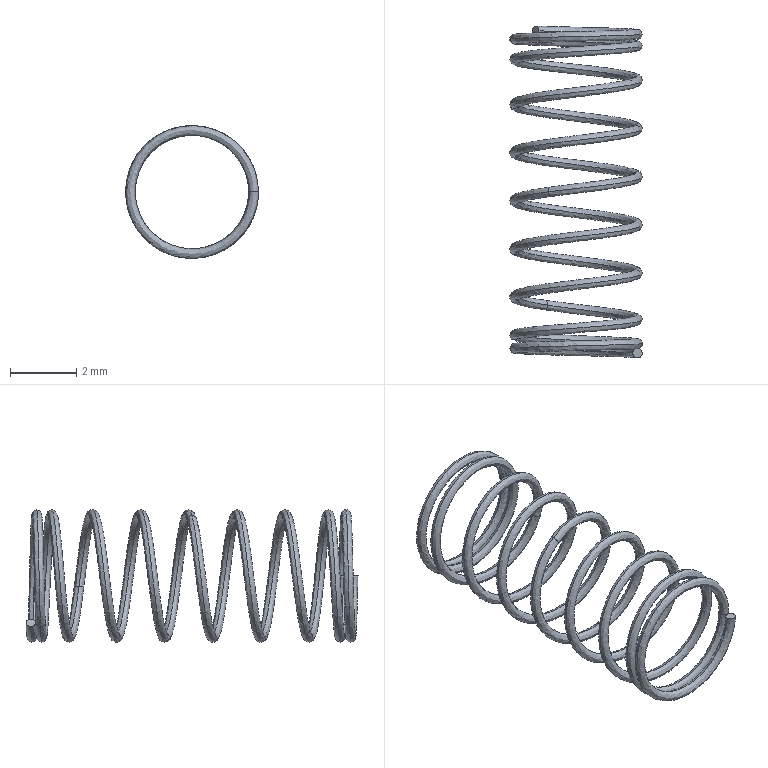Component | SolidWorks | CompressionSpringSpringConstant0.2-0.5D5L10-1 | 1 solid | 14 faces | volume 7 mm3 | spline 12 | plane 2